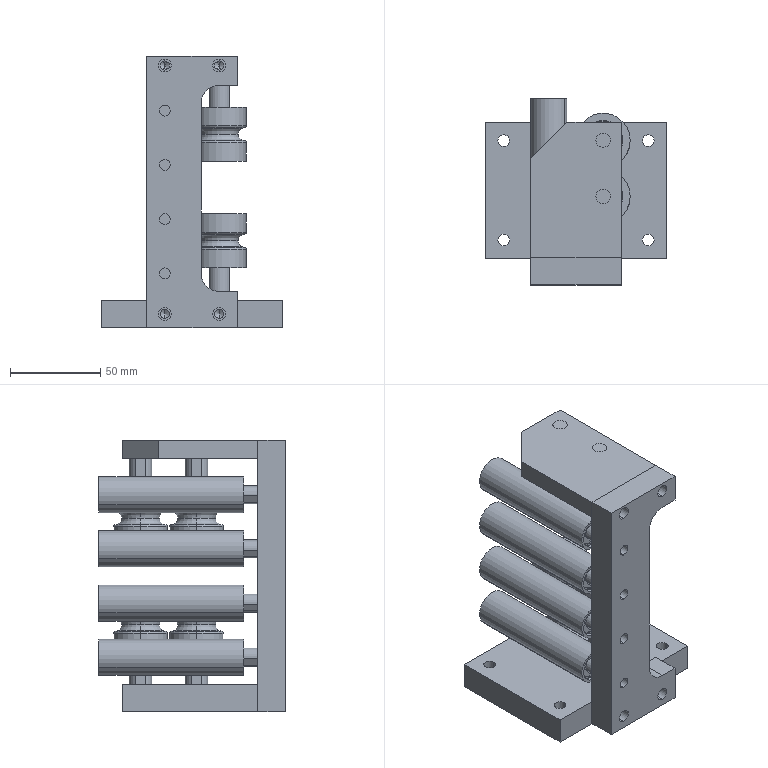Assembly | SolidWorks | mm | 43 component files | 43 solids | 977 faces | box 100 x 103 x 150 mm | volume 355258 mm3 | cylinder 522 | plane 271 | torus 160 | cone 24 | commonest cylinder face diameters 8 x48 6 x48 12.2 x32 19.3 x32 22 x32 8.6 x32 15 x32 17 x32
Bill of materials:
B608ZZ | 8 |  | Short annular cylinder (thick ring) with a central through bore; one end face carries two concentric narrow circular grooves dividing it into inner, middle and outer annular zones; opposite face appears plain; edges slightly rounded.
GB_T894-2017[AxisElasticRetainingRingTypeA(d0_9)8] | 4 |  | Thin flat open ring of constant thickness with a radial gap; each side of the gap ends in a rounded lug containing a small round hole, with a small notch/neck where the lugs join the ring.
JL001-03-03-001 | 4 |  | Stepped cylindrical pin: long slender shank, a larger-diameter collar with two opposite flats, and a short end stub of shank-like diameter; small circumferential grooves near the shank top end and between the collar and the stub.
JL001-03-03-002 | 4 |  | Hollow cylindrical sleeve with a central through bore and a single external circumferential groove of rounded (concave) profile at mid-height, giving a spool/sheave-like silhouette; bore shows an internal step.
B606ZZ | 8 |  | Short annular cylinder with central through bore and concentric circular grooves on its end face, nearly identical in form to unnamed part but shown in a different orientation.
GB_T894-2017[AxisElasticRetainingRingTypeA(d0_9)6] | 4 |  | Thin flat open ring with a radial gap flanked by two rounded lugs each with a small hole; similar in form to unnamed part, shown in a different orientation.
JL001-03-06-001 | 4 |  | Long slender stepped pin: long main shank, a short larger-diameter collar near one end, and a short stub beyond the collar; small grooves near the far shank end and next to the collar.
JL001-03-06-002 | 4 |  | Plain thin-walled straight round tube of constant outer and inner diameter, square-cut ends.
JL001-05-05-001 | 1 |  | Flat plate with C-shaped outline: a long spine with two end tabs, leaving a rectangular cutout on one side with filleted inner corners; eight round through holes (two at each tab end, four along the spine).
JL001-05-05-002 | 1 |  | Rectangular plate block with one corner cut off by a 45-degree chamfer; two through holes in the main face near one long edge and two drilled holes in one edge face.
JL001-05-05-003 | 1 |  | Rectangular flat plate with six through holes in the main face (four smaller corner holes and two larger holes, one near an edge and one central) plus two small blind holes in one edge face.
Mates:
1. coincident | JL001-05-05-003-1 face at (0, 0, 7.5) dir (0, 0, 1) | JL001-03-03-1/JL001-03-03-001-1 face at (15, 21.25, 7.5) dir (0, 0, -1)
2. coincident | JL001-05-05-003-1 face at (0, 0, 7.5) dir (0, 0, 1) | JL001-03-03-2/JL001-03-03-001-1 face at (15, -9.75, 7.5) dir (0, 0, -1)
3. coincident | JL001-03-06-5/JL001-03-06-001-1 face at (-17.735, -37.5, 86.686) dir (0, -1, 0) | JL001-05-05-001-1 face at (0, -37.5, 67.5) dir (0, 1, 0)
4. coincident | JL001-03-06-4/JL001-03-06-001-1 face at (-17.735, -37.5, 116.686) dir (0, -1, 0) | JL001-05-05-001-1 face at (0, -37.5, 67.5) dir (0, 1, 0)
5. concentric | JL001-05-05-003-1 face at (15, 27.5, 7.5) dir (0, 0, 1) r 4 | JL001-03-03-1/JL001-03-03-001-1 face at (15, 27.5, -2.5) dir (0, 0, -1) r 4
6. concentric | JL001-05-05-003-1 face at (15, -3.5, 7.5) dir (0, 0, 1) r 4 | JL001-03-03-2/JL001-03-03-001-1 face at (15, -3.5, -2.5) dir (0, 0, -1) r 4
7. concentric | JL001-05-05-001-1 face at (-15, -37.5, 82.5) dir (0, 1, 0) r 3 | JL001-03-06-5/JL001-03-06-001-1 face at (-15, -47.5, 82.5) dir (0, -1, 0) r 3
8. concentric | JL001-05-05-001-1 face at (-15, -37.5, 112.5) dir (0, 1, 0) r 3 | JL001-03-06-4/JL001-03-06-001-1 face at (-15, -47.5, 112.5) dir (0, -1, 0) r 3
9. coincident | JL001-05-05-003-1 face at (-50, -37.5, 7.5) dir (0, -1, 0) | JL001-05-05-001-1 face at (0, -37.5, 67.5) dir (0, 1, 0)
10. coincident | JL001-05-05-001-1 face at (0, -37.5, 67.5) dir (0, 1, 0) | JL001-05-05-002-1 face at (-25, -37.5, 142.5) dir (0, -1, 0)
11. coincident | JL001-05-05-001-1 face at (25, -37.5, -7.5) dir (1, 0, 0) | JL001-05-05-002-1 face at (25, 37.5, 142.5) dir (1, 0, 0)
12. coincident | JL001-05-05-001-1 face at (-25, -37.5, 142.5) dir (0, 0, 1) | JL001-05-05-002-1 face at (0, 0, 142.5) dir (0, 0, 1)
13. concentric | JL001-05-05-002-1 face at (15, -3.5, 142.5) dir (0, 0, 1) r 4 | JL001-03-03-4/JL001-03-03-001-1 face at (15, -3.5, 142.5) dir (0, 0, 1) r 4
14. concentric | JL001-05-05-002-1 face at (15, 27.5, 142.5) dir (0, 0, 1) r 4 | JL001-03-03-3/JL001-03-03-001-1 face at (15, 27.5, 142.5) dir (0, 0, 1) r 4
15. coincident | JL001-05-05-002-1 face at (0, 0, 132.5) dir (0, 0, -1) | JL001-03-03-3/JL001-03-03-001-1 face at (15, 33.75, 132.5) dir (0, 0, 1)
16. coincident | JL001-05-05-002-1 face at (0, 0, 132.5) dir (0, 0, -1) | JL001-03-03-4/JL001-03-03-001-1 face at (15, 2.75, 132.5) dir (0, 0, 1)
17. coincident | JL001-05-05-001-1 face at (0, -37.5, 67.5) dir (0, 1, 0) | JL001-03-06-6/JL001-03-06-001-1 face at (-17.735, -37.5, 56.686) dir (0, -1, 0)
18. coincident | JL001-05-05-001-1 face at (0, -37.5, 67.5) dir (0, 1, 0) | JL001-03-06-7/JL001-03-06-001-1 face at (-17.735, -37.5, 26.686) dir (0, -1, 0)
19. concentric | JL001-05-05-001-1 face at (-15, -37.5, 52.5) dir (0, 1, 0) r 3 | JL001-03-06-6/JL001-03-06-001-1 face at (-15, -47.5, 52.5) dir (0, -1, 0) r 3
20. concentric | JL001-05-05-001-1 face at (-15, -37.5, 22.5) dir (0, 1, 0) r 3 | JL001-03-06-7/JL001-03-06-001-1 face at (-15, -47.5, 22.5) dir (0, -1, 0) r 3
21. concentric | JL001-05-05-003-1 face at (-15, -37.5, 0) dir (0, -1, 0) r 2.5 | JL001-05-05-001-1 face at (-15, -37.5, 0) dir (0, 1, 0) r 3.5
22. concentric | JL001-05-05-003-1 face at (15, -37.5, 0) dir (0, -1, 0) r 2.5 | JL001-05-05-001-1 face at (15, -37.5, 0) dir (0, 1, 0) r 3.5
23. coincident | JL001-03-03-1/JL001-03-03-001-1 face at (20.5, 37.35, -2.5) dir (1, 0, 0) | JL001-03-03-2/JL001-03-03-001-1 face at (20.5, 6.35, -2.5) dir (1, 0, 0)
24. coincident | JL001-03-03-3/JL001-03-03-001-1 face at (20.5, 17.65, 142.5) dir (1, 0, 0) | JL001-03-03-4/JL001-03-03-001-1 face at (20.5, -13.35, 142.5) dir (1, 0, 0)
25. concentric | JL001-03-03-001-1 face at (0, 0, 0) dir (0, -1, 0) r 4 | B608ZZ-1 face at (0, 30.3, 0) dir (0, 1, 0) r 4
26. coincident | JL001-03-03-001-1 face at (4, 30, 0) dir (0, 1, 0) | B608ZZ-1 face at (4.3, 30, 0) dir (0, -1, 0)
27. concentric | B608ZZ-1 face at (0, 30.3, 0) dir (0, 1, 0) r 11 | JL001-03-03-002-1 face at (0, 43, 0) dir (0, 1, 0) r 11
28. coincident | B608ZZ-1 face at (10.7, 37, 0) dir (0, 1, 0) | JL001-03-03-002-1 face at (11, 37, 0) dir (0, -1, 0)
29. concentric | JL001-03-03-001-1 face at (0, 0, 0) dir (0, -1, 0) r 4 | B608ZZ-2 face at (0, 49.3, 0) dir (0, 1, 0) r 4
30. coincident | JL001-03-03-002-1 face at (9, 49, 0) dir (0, 1, 0) | B608ZZ-2 face at (9.65, 49, 0) dir (0, -1, 0)
31. concentric | JL001-03-03-001-1 face at (0, 0, 0) dir (0, -1, 0) r 3.7 | GB_T894-2017[AxisElasticRetainingRingTypeA(d0_9)8]-1 face at (0, 56, 0) dir (0, 1, 0) r 3.7
32. coincident | JL001-03-03-001-1 face at (3.7, 56, 0) dir (0, 1, 0) | GB_T894-2017[AxisElasticRetainingRingTypeA(d0_9)8]-1 face at (-0.6, 56, -5.251) dir (0, -1, 0)
33. concentric | JL001-03-06-001-1 face at (0, 0, 0) dir (0, -1, 0) r 3 | B606ZZ-1 face at (0, 20.3, 0) dir (0, 1, 0) r 3
34. coincident | JL001-03-06-001-1 face at (3, 20, 0) dir (0, 1, 0) | B606ZZ-1 face at (3.3, 20, 0) dir (0, -1, 0)
35. concentric | B606ZZ-1 face at (0, 20.3, 0) dir (0, 1, 0) r 8.5 | JL001-03-06-002-1 face at (0, 98, 0) dir (0, 1, 0) r 8.5
36. coincident | B606ZZ-1 face at (8.2, 26, 0) dir (0, 1, 0) | JL001-03-06-002-1 face at (8.5, 26, 0) dir (0, -1, 0)
37. concentric | JL001-03-06-001-1 face at (0, 0, 0) dir (0, -1, 0) r 3 | B606ZZ-2 face at (0, 90.3, 0) dir (0, 1, 0) r 3
38. coincident | JL001-03-06-002-1 face at (7, 90, 0) dir (0, 1, 0) | B606ZZ-2 face at (7.5, 90, 0) dir (0, -1, 0)
39. concentric | JL001-03-06-001-1 face at (0, 0, 0) dir (0, -1, 0) r 2.8 | GB_T894-2017[AxisElasticRetainingRingTypeA(d0_9)6]-1 face at (0, 96, 0) dir (0, 1, 0) r 2.8
40. coincident | JL001-03-06-001-1 face at (2.8, 96, 0) dir (0, 1, 0) | GB_T894-2017[AxisElasticRetainingRingTypeA(d0_9)6]-1 face at (0.7337, 96, 4.063) dir (0, -1, 0)